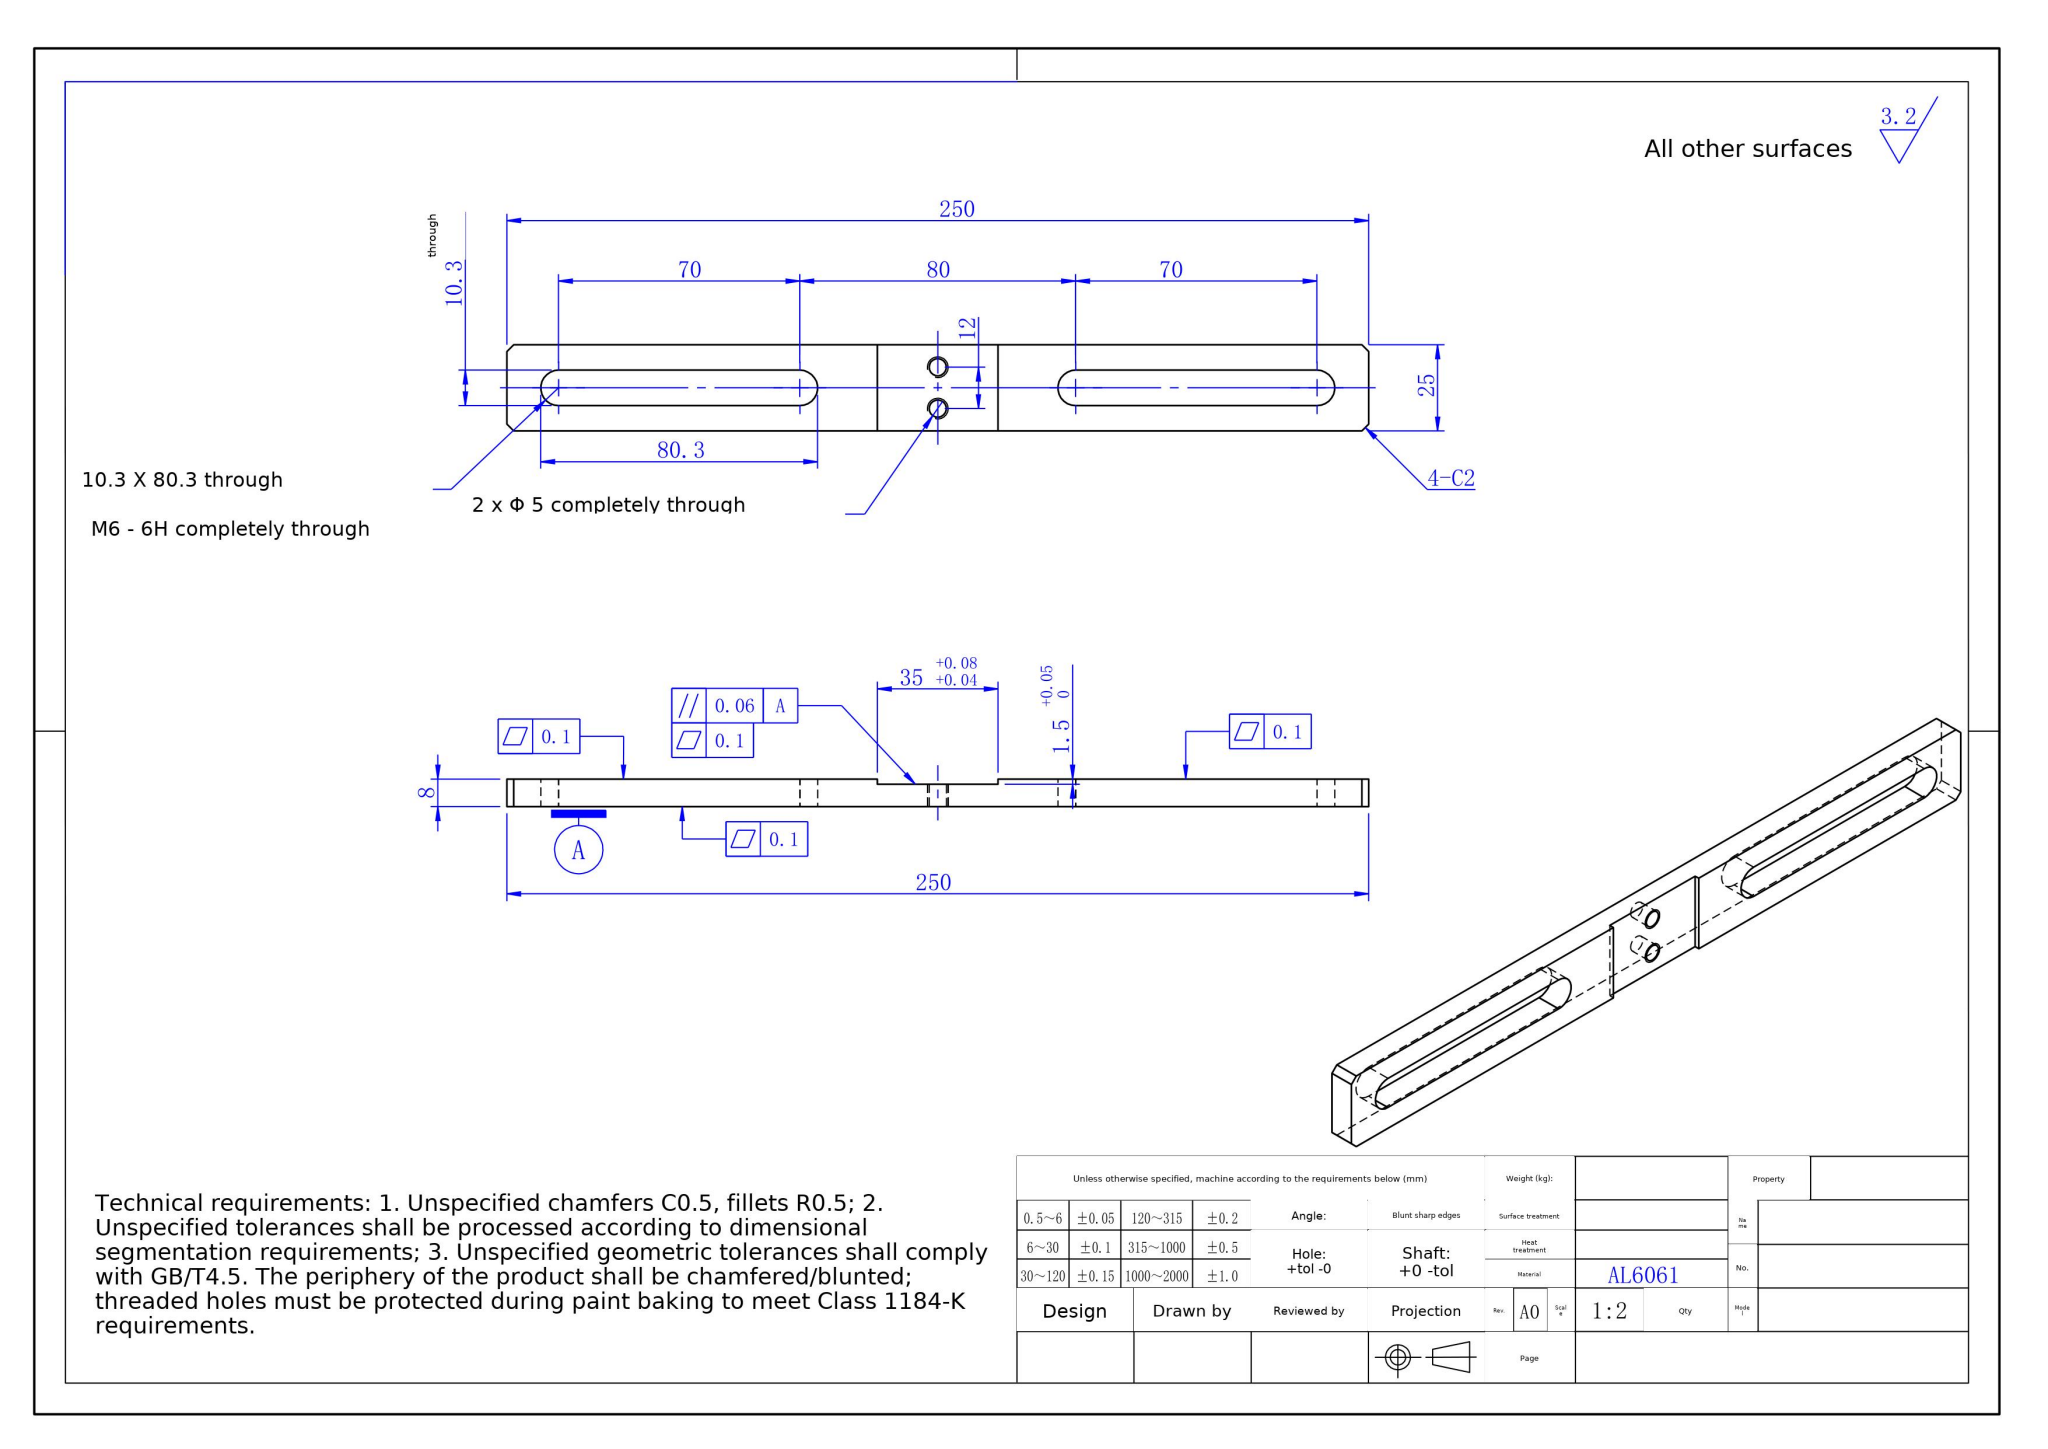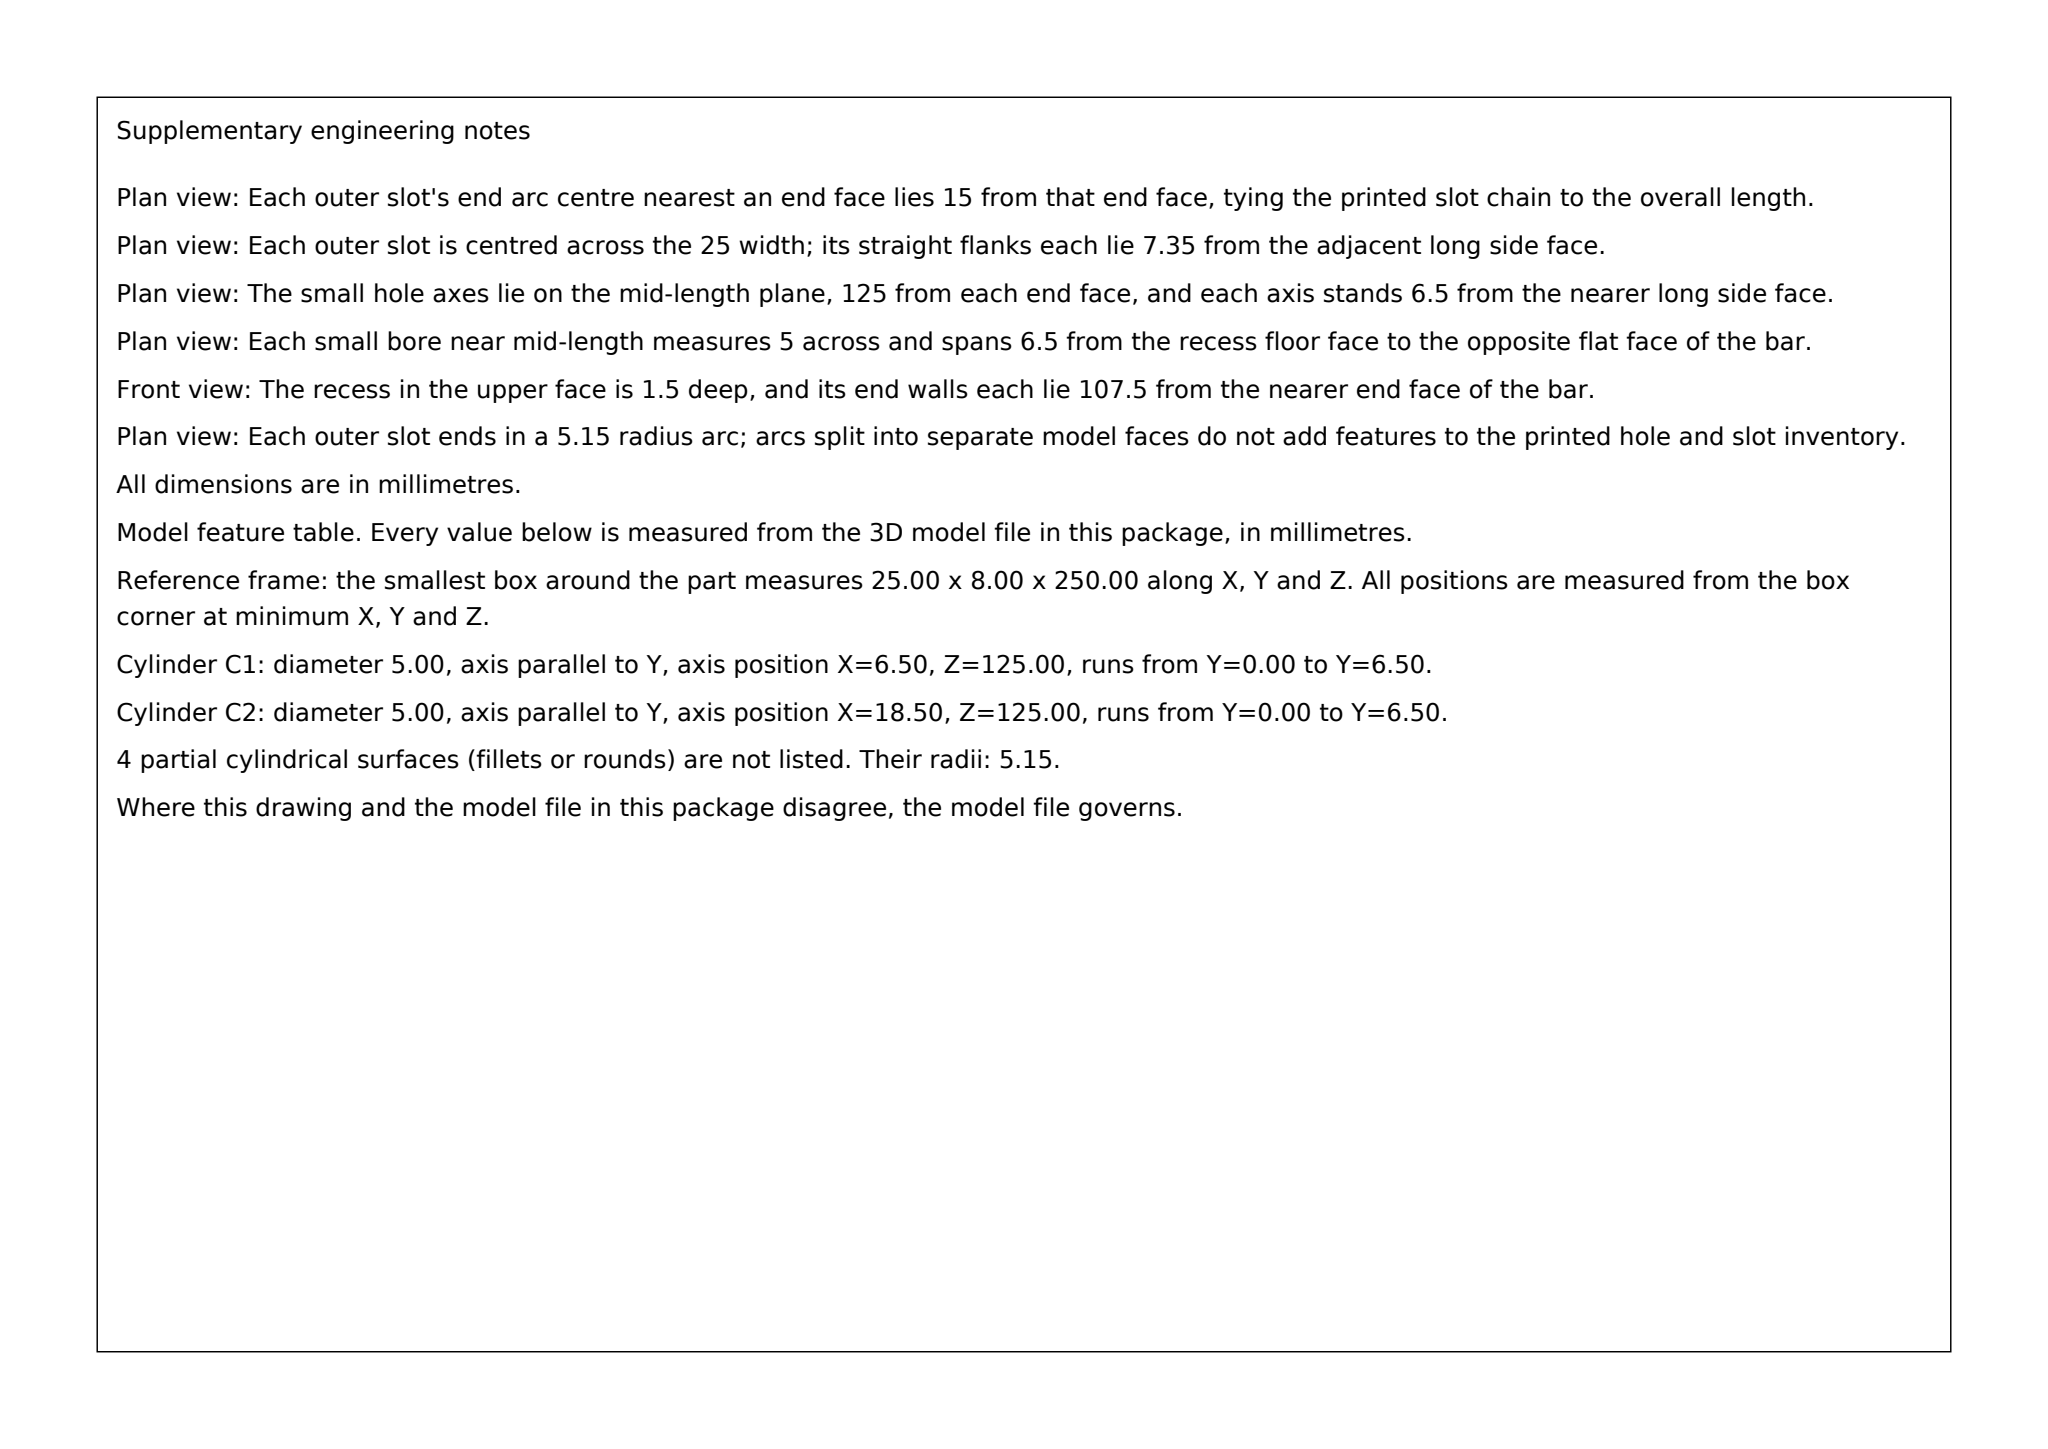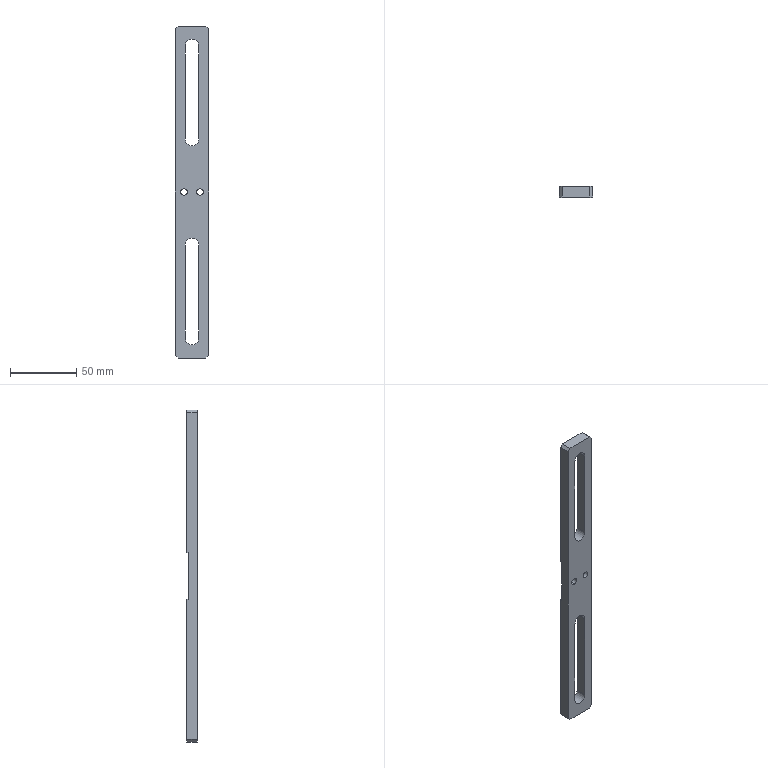Part | SolidWorks | mm | 1 solid | 28 faces | box 25 x 8 x 250 mm | volume 35499 mm3 | plane 18 | cylinder 10 | commonest cylinder face diameters 10.3 x6 5 x4
build123d program:
from build123d import *

# Parameters (mm, degrees)
SKETCH1_W           = 25
SKETCH1_H           = 250
BOSS_EXTRUDE1_DEPTH = 8
SKETCH2_W           = 25
SKETCH2_H           = 35
CUT_EXTRUDE1_DEPTH  = 1.5
M6_TAPPED_HOLE1_D   = 5
CUT_EXTRUDE2_DEPTH  = 10
CHAMFER1_SIZE       = 2


with BuildPart() as part:
    # Sketch1 → Boss-Extrude1 (new body)
    with BuildSketch(Plane(origin=(0, 0, 0), x_dir=(1, 0, 0), z_dir=(0, 1, 0))):
        Rectangle(SKETCH1_W, SKETCH1_H)
    extrude(amount=BOSS_EXTRUDE1_DEPTH)

    # Sketch2 → Cut-Extrude1 (cut)
    with BuildSketch(Plane(origin=(0, 8, 0), x_dir=(1, 0, 0), z_dir=(0, 1, 0))):
        Rectangle(SKETCH2_W, SKETCH2_H)
    extrude(amount=-CUT_EXTRUDE1_DEPTH, mode=Mode.SUBTRACT)

    # M6 Tapped Hole1 (through all)
    with Locations(Plane(origin=(0, 6.5, 0), x_dir=(1, 0, 0), z_dir=(0, 1, 0))):
        with Locations((-6, 0), (6, 0)):
            Hole(M6_TAPPED_HOLE1_D / 2)

    # Sketch5 → Cut-Extrude2 (cut)
    with BuildSketch(Plane(origin=(0, 8, 0), x_dir=(1, 0, 0), z_dir=(0, 1, 0))):
        with BuildLine():
            Line((5.15, -40), (5.15, -110))
            ThreePointArc((5.15, -110), (0, -115.15), (-5.15, -110))
            Line((-5.15, -110), (-5.15, -40))
            ThreePointArc((-5.15, -40), (0, -34.85), (5.15, -40))
        make_face()
        with BuildLine():
            Line((5.15, 40), (5.15, 110))
            ThreePointArc((5.15, 110), (0, 115.15), (-5.15, 110))
            Line((-5.15, 110), (-5.15, 40))
            ThreePointArc((-5.15, 40), (0, 34.85), (5.15, 40))
        make_face()
    extrude(amount=-CUT_EXTRUDE2_DEPTH, mode=Mode.SUBTRACT)

    # Chamfer1
    chamfer1_edges = [part.edges().sort_by_distance(p)[0] for p in [
        (12.5, 4, 125),
        (-12.5, 4, 125),
        (-12.5, 4, -125),
        (12.5, 4, -125),
    ]]
    chamfer(chamfer1_edges, length=CHAMFER1_SIZE)


solid = part.part
STEP:
#1=CARTESIAN_POINT('',(0.,0.,115.15));
#2=VERTEX_POINT('',#1);
#3=CARTESIAN_POINT('',(5.15,0.,110.));
#4=VERTEX_POINT('',#3);
#5=CARTESIAN_POINT('',(0.,0.,110.));
#6=DIRECTION('',(0.,1.,0.));
#7=DIRECTION('',(0.,0.,1.));
#8=AXIS2_PLACEMENT_3D('',#5,#6,#7);
#9=CIRCLE('',#8,5.15);
#10=EDGE_CURVE('',#2,#4,#9,.T.);
#11=ORIENTED_EDGE('',*,*,#10,.F.);
#12=CARTESIAN_POINT('',(0.,8.,115.15));
#13=VERTEX_POINT('',#12);
#14=CARTESIAN_POINT('',(0.,-2.,115.15));
#15=DIRECTION('',(0.,1.,0.));
#16=VECTOR('',#15,1000.);
#17=LINE('',#14,#16);
#18=EDGE_CURVE('',#2,#13,#17,.T.);
#19=ORIENTED_EDGE('',*,*,#18,.T.);
#20=CARTESIAN_POINT('',(5.15,8.,110.));
#21=VERTEX_POINT('',#20);
#22=CARTESIAN_POINT('',(0.,8.,110.));
#23=DIRECTION('',(0.,1.,0.));
#24=DIRECTION('',(0.,0.,1.));
#25=AXIS2_PLACEMENT_3D('',#22,#23,#24);
#26=CIRCLE('',#25,5.15);
#27=EDGE_CURVE('',#13,#21,#26,.T.);
#28=ORIENTED_EDGE('',*,*,#27,.T.);
#29=CARTESIAN_POINT('',(5.15,-2.,110.));
#30=DIRECTION('',(0.,1.,0.));
#31=VECTOR('',#30,1000.);
#32=LINE('',#29,#31);
#33=EDGE_CURVE('',#4,#21,#32,.T.);
#34=ORIENTED_EDGE('',*,*,#33,.F.);
#35=EDGE_LOOP('',(#11,#19,#28,#34));
#36=FACE_OUTER_BOUND('',#35,.T.);
#37=CARTESIAN_POINT('',(0.,-2.,110.));
#38=DIRECTION('',(0.,1.,0.));
#39=DIRECTION('',(0.,0.,1.));
#40=AXIS2_PLACEMENT_3D('',#37,#38,#39);
#41=CYLINDRICAL_SURFACE('',#40,5.15);
#42=ADVANCED_FACE('',(#36),#41,.F.);
#43=CARTESIAN_POINT('',(-0.,0.,-34.85));
#44=VERTEX_POINT('',#43);
#45=CARTESIAN_POINT('',(5.15,0.,-40.));
#46=VERTEX_POINT('',#45);
#47=CARTESIAN_POINT('',(-0.,0.,-40.));
#48=DIRECTION('',(0.,1.,0.));
#49=DIRECTION('',(0.,0.,1.));
#50=AXIS2_PLACEMENT_3D('',#47,#48,#49);
#51=CIRCLE('',#50,5.15);
#52=EDGE_CURVE('',#44,#46,#51,.T.);
#53=ORIENTED_EDGE('',*,*,#52,.F.);
#54=CARTESIAN_POINT('',(-0.,8.,-34.85));
#55=VERTEX_POINT('',#54);
#56=CARTESIAN_POINT('',(-0.,-2.,-34.85));
#57=DIRECTION('',(0.,1.,0.));
#58=VECTOR('',#57,1000.);
#59=LINE('',#56,#58);
#60=EDGE_CURVE('',#44,#55,#59,.T.);
#61=ORIENTED_EDGE('',*,*,#60,.T.);
#62=CARTESIAN_POINT('',(5.15,8.,-40.));
#63=VERTEX_POINT('',#62);
#64=CARTESIAN_POINT('',(-0.,8.,-40.));
#65=DIRECTION('',(0.,1.,0.));
#66=DIRECTION('',(0.,0.,-1.));
#67=AXIS2_PLACEMENT_3D('',#64,#65,#66);
#68=CIRCLE('',#67,5.15);
#69=EDGE_CURVE('',#55,#63,#68,.T.);
#70=ORIENTED_EDGE('',*,*,#69,.T.);
#71=CARTESIAN_POINT('',(5.15,-2.,-40.));
#72=DIRECTION('',(0.,1.,0.));
#73=VECTOR('',#72,1000.);
#74=LINE('',#71,#73);
#75=EDGE_CURVE('',#46,#63,#74,.T.);
#76=ORIENTED_EDGE('',*,*,#75,.F.);
#77=EDGE_LOOP('',(#53,#61,#70,#76));
#78=FACE_OUTER_BOUND('',#77,.T.);
#79=CARTESIAN_POINT('',(-0.,-2.,-40.));
#80=DIRECTION('',(0.,1.,0.));
#81=DIRECTION('',(0.,0.,1.));
#82=AXIS2_PLACEMENT_3D('',#79,#80,#81);
#83=CYLINDRICAL_SURFACE('',#82,5.15);
#84=ADVANCED_FACE('',(#78),#83,.F.);
#85=CARTESIAN_POINT('',(-6.,0.,-2.5));
#86=VERTEX_POINT('',#85);
#87=CARTESIAN_POINT('',(-6.,0.,2.5));
#88=VERTEX_POINT('',#87);
#89=CARTESIAN_POINT('',(-6.,0.,0.));
#90=DIRECTION('',(0.,1.,0.));
#91=DIRECTION('',(0.,0.,1.));
#92=AXIS2_PLACEMENT_3D('',#89,#90,#91);
#93=CIRCLE('',#92,2.5);
#94=EDGE_CURVE('',#86,#88,#93,.T.);
#95=ORIENTED_EDGE('',*,*,#94,.F.);
#96=CARTESIAN_POINT('',(-6.,6.5,-2.5));
#97=VERTEX_POINT('',#96);
#98=CARTESIAN_POINT('',(-6.,6.5,-2.5));
#99=DIRECTION('',(0.,1.,0.));
#100=VECTOR('',#99,1000.);
#101=LINE('',#98,#100);
#102=EDGE_CURVE('',#86,#97,#101,.T.);
#103=ORIENTED_EDGE('',*,*,#102,.T.);
#104=CARTESIAN_POINT('',(-6.,6.5,2.5));
#105=VERTEX_POINT('',#104);
#106=CARTESIAN_POINT('',(-6.,6.5,0.));
#107=DIRECTION('',(0.,1.,0.));
#108=DIRECTION('',(0.,0.,1.));
#109=AXIS2_PLACEMENT_3D('',#106,#107,#108);
#110=CIRCLE('',#109,2.5);
#111=EDGE_CURVE('',#97,#105,#110,.T.);
#112=ORIENTED_EDGE('',*,*,#111,.T.);
#113=CARTESIAN_POINT('',(-6.,6.5,2.5));
#114=DIRECTION('',(0.,1.,0.));
#115=VECTOR('',#114,1000.);
#116=LINE('',#113,#115);
#117=EDGE_CURVE('',#88,#105,#116,.T.);
#118=ORIENTED_EDGE('',*,*,#117,.F.);
#119=EDGE_LOOP('',(#95,#103,#112,#118));
#120=FACE_OUTER_BOUND('',#119,.T.);
#121=CARTESIAN_POINT('',(-6.,6.5,0.));
#122=DIRECTION('',(0.,1.,0.));
#123=DIRECTION('',(0.,0.,1.));
#124=AXIS2_PLACEMENT_3D('',#121,#122,#123);
#125=CYLINDRICAL_SURFACE('',#124,2.5);
#126=ADVANCED_FACE('',(#120),#125,.F.);
#127=CARTESIAN_POINT('',(6.,0.,-2.5));
#128=VERTEX_POINT('',#127);
#129=CARTESIAN_POINT('',(6.,0.,2.5));
#130=VERTEX_POINT('',#129);
#131=CARTESIAN_POINT('',(6.,0.,0.));
#132=DIRECTION('',(0.,1.,0.));
#133=DIRECTION('',(0.,0.,1.));
#134=AXIS2_PLACEMENT_3D('',#131,#132,#133);
#135=CIRCLE('',#134,2.5);
#136=EDGE_CURVE('',#128,#130,#135,.T.);
#137=ORIENTED_EDGE('',*,*,#136,.F.);
#138=CARTESIAN_POINT('',(6.,6.5,-2.5));
#139=VERTEX_POINT('',#138);
#140=CARTESIAN_POINT('',(6.,6.5,-2.5));
#141=DIRECTION('',(0.,1.,0.));
#142=VECTOR('',#141,1000.);
#143=LINE('',#140,#142);
#144=EDGE_CURVE('',#128,#139,#143,.T.);
#145=ORIENTED_EDGE('',*,*,#144,.T.);
#146=CARTESIAN_POINT('',(6.,6.5,2.5));
#147=VERTEX_POINT('',#146);
#148=CARTESIAN_POINT('',(6.,6.5,0.));
#149=DIRECTION('',(0.,1.,0.));
#150=DIRECTION('',(0.,0.,1.));
#151=AXIS2_PLACEMENT_3D('',#148,#149,#150);
#152=CIRCLE('',#151,2.5);
#153=EDGE_CURVE('',#139,#147,#152,.T.);
#154=ORIENTED_EDGE('',*,*,#153,.T.);
#155=CARTESIAN_POINT('',(6.,6.5,2.5));
#156=DIRECTION('',(0.,1.,0.));
#157=VECTOR('',#156,1000.);
#158=LINE('',#155,#157);
#159=EDGE_CURVE('',#130,#147,#158,.T.);
#160=ORIENTED_EDGE('',*,*,#159,.F.);
#161=EDGE_LOOP('',(#137,#145,#154,#160));
#162=FACE_OUTER_BOUND('',#161,.T.);
#163=CARTESIAN_POINT('',(6.,6.5,0.));
#164=DIRECTION('',(0.,1.,0.));
#165=DIRECTION('',(0.,0.,1.));
#166=AXIS2_PLACEMENT_3D('',#163,#164,#165);
#167=CYLINDRICAL_SURFACE('',#166,2.5);
#168=ADVANCED_FACE('',(#162),#167,.F.);
#169=CARTESIAN_POINT('',(5.15,8.,40.));
#170=VERTEX_POINT('',#169);
#171=CARTESIAN_POINT('',(-5.15,8.,40.));
#172=VERTEX_POINT('',#171);
#173=CARTESIAN_POINT('',(0.,8.,40.));
#174=DIRECTION('',(0.,1.,0.));
#175=DIRECTION('',(0.,0.,1.));
#176=AXIS2_PLACEMENT_3D('',#173,#174,#175);
#177=CIRCLE('',#176,5.15);
#178=EDGE_CURVE('',#170,#172,#177,.T.);
#179=ORIENTED_EDGE('',*,*,#178,.F.);
#180=CARTESIAN_POINT('',(5.15,8.,40.));
#181=DIRECTION('',(-0.,0.,-1.));
#182=VECTOR('',#181,1000.);
#183=LINE('',#180,#182);
#184=EDGE_CURVE('',#21,#170,#183,.T.);
#185=ORIENTED_EDGE('',*,*,#184,.F.);
#186=ORIENTED_EDGE('',*,*,#27,.F.);
#187=CARTESIAN_POINT('',(-5.15,8.,110.));
#188=VERTEX_POINT('',#187);
#189=CARTESIAN_POINT('',(0.,8.,110.));
#190=DIRECTION('',(0.,1.,0.));
#191=DIRECTION('',(0.,0.,1.));
#192=AXIS2_PLACEMENT_3D('',#189,#190,#191);
#193=CIRCLE('',#192,5.15);
#194=EDGE_CURVE('',#188,#13,#193,.T.);
#195=ORIENTED_EDGE('',*,*,#194,.F.);
#196=CARTESIAN_POINT('',(-5.15,8.,40.));
#197=DIRECTION('',(-0.,0.,1.));
#198=VECTOR('',#197,1000.);
#199=LINE('',#196,#198);
#200=EDGE_CURVE('',#172,#188,#199,.T.);
#201=ORIENTED_EDGE('',*,*,#200,.F.);
#202=EDGE_LOOP('',(#179,#185,#186,#195,#201));
#203=FACE_BOUND('',#202,.T.);
#204=CARTESIAN_POINT('',(-12.5,8.,17.5));
#205=VERTEX_POINT('',#204);
#206=CARTESIAN_POINT('',(-12.5,8.,123.));
#207=VERTEX_POINT('',#206);
#208=CARTESIAN_POINT('',(-12.5,8.,-125.));
#209=DIRECTION('',(0.,0.,1.));
#210=VECTOR('',#209,1000.);
#211=LINE('',#208,#210);
#212=EDGE_CURVE('',#205,#207,#211,.T.);
#213=ORIENTED_EDGE('',*,*,#212,.T.);
#214=CARTESIAN_POINT('',(-10.5,8.,125.));
#215=VERTEX_POINT('',#214);
#216=CARTESIAN_POINT('',(-67.75,8.,67.75));
#217=DIRECTION('',(0.7071,0.,0.7071));
#218=VECTOR('',#217,1000.);
#219=LINE('',#216,#218);
#220=EDGE_CURVE('',#207,#215,#219,.T.);
#221=ORIENTED_EDGE('',*,*,#220,.T.);
#222=CARTESIAN_POINT('',(10.5,8.,125.));
#223=VERTEX_POINT('',#222);
#224=CARTESIAN_POINT('',(-12.5,8.,125.));
#225=DIRECTION('',(1.,0.,0.));
#226=VECTOR('',#225,1000.);
#227=LINE('',#224,#226);
#228=EDGE_CURVE('',#215,#223,#227,.T.);
#229=ORIENTED_EDGE('',*,*,#228,.T.);
#230=CARTESIAN_POINT('',(12.5,8.,123.));
#231=VERTEX_POINT('',#230);
#232=CARTESIAN_POINT('',(67.75,8.,67.75));
#233=DIRECTION('',(0.7071,0.,-0.7071));
#234=VECTOR('',#233,1000.);
#235=LINE('',#232,#234);
#236=EDGE_CURVE('',#223,#231,#235,.T.);
#237=ORIENTED_EDGE('',*,*,#236,.T.);
#238=CARTESIAN_POINT('',(12.5,8.,17.5));
#239=VERTEX_POINT('',#238);
#240=CARTESIAN_POINT('',(12.5,8.,-125.));
#241=DIRECTION('',(-0.,0.,-1.));
#242=VECTOR('',#241,1000.);
#243=LINE('',#240,#242);
#244=EDGE_CURVE('',#231,#239,#243,.T.);
#245=ORIENTED_EDGE('',*,*,#244,.T.);
#246=CARTESIAN_POINT('',(-12.5,8.,17.5));
#247=DIRECTION('',(1.,0.,0.));
#248=VECTOR('',#247,1000.);
#249=LINE('',#246,#248);
#250=EDGE_CURVE('',#205,#239,#249,.T.);
#251=ORIENTED_EDGE('',*,*,#250,.F.);
#252=EDGE_LOOP('',(#213,#221,#229,#237,#245,#251));
#253=FACE_OUTER_BOUND('',#252,.T.);
#254=CARTESIAN_POINT('',(0.,8.,0.));
#255=DIRECTION('',(0.,1.,0.));
#256=DIRECTION('',(0.,0.,1.));
#257=AXIS2_PLACEMENT_3D('',#254,#255,#256);
#258=PLANE('',#257);
#259=ADVANCED_FACE('',(#203,#253),#258,.T.);
#260=CARTESIAN_POINT('',(12.5,0.,123.));
#261=VERTEX_POINT('',#260);
#262=CARTESIAN_POINT('',(12.5,0.,-123.));
#263=VERTEX_POINT('',#262);
#264=CARTESIAN_POINT('',(12.5,0.,-125.));
#265=DIRECTION('',(-0.,0.,-1.));
#266=VECTOR('',#265,1000.);
#267=LINE('',#264,#266);
#268=EDGE_CURVE('',#261,#263,#267,.T.);
#269=ORIENTED_EDGE('',*,*,#268,.T.);
#270=CARTESIAN_POINT('',(12.5,8.,-123.));
#271=VERTEX_POINT('',#270);
#272=CARTESIAN_POINT('',(12.5,8.,-123.));
#273=DIRECTION('',(0.,1.,0.));
#274=VECTOR('',#273,1000.);
#275=LINE('',#272,#274);
#276=EDGE_CURVE('',#263,#271,#275,.T.);
#277=ORIENTED_EDGE('',*,*,#276,.T.);
#278=CARTESIAN_POINT('',(12.5,8.,-17.5));
#279=VERTEX_POINT('',#278);
#280=CARTESIAN_POINT('',(12.5,8.,-125.));
#281=DIRECTION('',(-0.,0.,-1.));
#282=VECTOR('',#281,1000.);
#283=LINE('',#280,#282);
#284=EDGE_CURVE('',#279,#271,#283,.T.);
#285=ORIENTED_EDGE('',*,*,#284,.F.);
#286=CARTESIAN_POINT('',(12.5,6.5,-17.5));
#287=VERTEX_POINT('',#286);
#288=CARTESIAN_POINT('',(12.5,6.5,-17.5));
#289=DIRECTION('',(0.,1.,0.));
#290=VECTOR('',#289,1000.);
#291=LINE('',#288,#290);
#292=EDGE_CURVE('',#287,#279,#291,.T.);
#293=ORIENTED_EDGE('',*,*,#292,.F.);
#294=CARTESIAN_POINT('',(12.5,6.5,17.5));
#295=VERTEX_POINT('',#294);
#296=CARTESIAN_POINT('',(12.5,6.5,-17.5));
#297=DIRECTION('',(0.,0.,-1.));
#298=VECTOR('',#297,1000.);
#299=LINE('',#296,#298);
#300=EDGE_CURVE('',#295,#287,#299,.T.);
#301=ORIENTED_EDGE('',*,*,#300,.F.);
#302=CARTESIAN_POINT('',(12.5,6.5,17.5));
#303=DIRECTION('',(0.,1.,0.));
#304=VECTOR('',#303,1000.);
#305=LINE('',#302,#304);
#306=EDGE_CURVE('',#295,#239,#305,.T.);
#307=ORIENTED_EDGE('',*,*,#306,.T.);
#308=ORIENTED_EDGE('',*,*,#244,.F.);
#309=CARTESIAN_POINT('',(12.5,8.,123.));
#310=DIRECTION('',(0.,-1.,0.));
#311=VECTOR('',#310,1000.);
#312=LINE('',#309,#311);
#313=EDGE_CURVE('',#231,#261,#312,.T.);
#314=ORIENTED_EDGE('',*,*,#313,.T.);
#315=EDGE_LOOP('',(#269,#277,#285,#293,#301,#307,#308,#314));
#316=FACE_OUTER_BOUND('',#315,.T.);
#317=CARTESIAN_POINT('',(12.5,8.,-125.));
#318=DIRECTION('',(-1.,0.,0.));
#319=DIRECTION('',(0.,0.,1.));
#320=AXIS2_PLACEMENT_3D('',#317,#318,#319);
#321=PLANE('',#320);
#322=ADVANCED_FACE('',(#316),#321,.F.);
#323=CARTESIAN_POINT('',(10.5,0.,-125.));
#324=VERTEX_POINT('',#323);
#325=CARTESIAN_POINT('',(-10.5,0.,-125.));
#326=VERTEX_POINT('',#325);
#327=CARTESIAN_POINT('',(-12.5,0.,-125.));
#328=DIRECTION('',(-1.,0.,0.));
#329=VECTOR('',#328,1000.);
#330=LINE('',#327,#329);
#331=EDGE_CURVE('',#324,#326,#330,.T.);
#332=ORIENTED_EDGE('',*,*,#331,.T.);
#333=CARTESIAN_POINT('',(-10.5,8.,-125.));
#334=VERTEX_POINT('',#333);
#335=CARTESIAN_POINT('',(-10.5,8.,-125.));
#336=DIRECTION('',(0.,1.,0.));
#337=VECTOR('',#336,1000.);
#338=LINE('',#335,#337);
#339=EDGE_CURVE('',#326,#334,#338,.T.);
#340=ORIENTED_EDGE('',*,*,#339,.T.);
#341=CARTESIAN_POINT('',(10.5,8.,-125.));
#342=VERTEX_POINT('',#341);
#343=CARTESIAN_POINT('',(-12.5,8.,-125.));
#344=DIRECTION('',(-1.,0.,0.));
#345=VECTOR('',#344,1000.);
#346=LINE('',#343,#345);
#347=EDGE_CURVE('',#342,#334,#346,.T.);
#348=ORIENTED_EDGE('',*,*,#347,.F.);
#349=CARTESIAN_POINT('',(10.5,8.,-125.));
#350=DIRECTION('',(0.,-1.,0.));
#351=VECTOR('',#350,1000.);
#352=LINE('',#349,#351);
#353=EDGE_CURVE('',#342,#324,#352,.T.);
#354=ORIENTED_EDGE('',*,*,#353,.T.);
#355=EDGE_LOOP('',(#332,#340,#348,#354));
#356=FACE_OUTER_BOUND('',#355,.T.);
#357=CARTESIAN_POINT('',(-12.5,8.,-125.));
#358=DIRECTION('',(0.,0.,1.));
#359=DIRECTION('',(1.,0.,0.));
#360=AXIS2_PLACEMENT_3D('',#357,#358,#359);
#361=PLANE('',#360);
#362=ADVANCED_FACE('',(#356),#361,.F.);
#363=CARTESIAN_POINT('',(-12.5,8.,-123.));
#364=VERTEX_POINT('',#363);
#365=CARTESIAN_POINT('',(-12.5,8.,-17.5));
#366=VERTEX_POINT('',#365);
#367=CARTESIAN_POINT('',(-12.5,8.,-125.));
#368=DIRECTION('',(0.,0.,1.));
#369=VECTOR('',#368,1000.);
#370=LINE('',#367,#369);
#371=EDGE_CURVE('',#364,#366,#370,.T.);
#372=ORIENTED_EDGE('',*,*,#371,.F.);
#373=CARTESIAN_POINT('',(-12.5,0.,-123.));
#374=VERTEX_POINT('',#373);
#375=CARTESIAN_POINT('',(-12.5,8.,-123.));
#376=DIRECTION('',(0.,-1.,0.));
#377=VECTOR('',#376,1000.);
#378=LINE('',#375,#377);
#379=EDGE_CURVE('',#364,#374,#378,.T.);
#380=ORIENTED_EDGE('',*,*,#379,.T.);
#381=CARTESIAN_POINT('',(-12.5,0.,123.));
#382=VERTEX_POINT('',#381);
#383=CARTESIAN_POINT('',(-12.5,0.,-125.));
#384=DIRECTION('',(0.,0.,1.));
#385=VECTOR('',#384,1000.);
#386=LINE('',#383,#385);
#387=EDGE_CURVE('',#374,#382,#386,.T.);
#388=ORIENTED_EDGE('',*,*,#387,.T.);
#389=CARTESIAN_POINT('',(-12.5,8.,123.));
#390=DIRECTION('',(0.,1.,0.));
#391=VECTOR('',#390,1000.);
#392=LINE('',#389,#391);
#393=EDGE_CURVE('',#382,#207,#392,.T.);
#394=ORIENTED_EDGE('',*,*,#393,.T.);
#395=ORIENTED_EDGE('',*,*,#212,.F.);
#396=CARTESIAN_POINT('',(-12.5,6.5,17.5));
#397=VERTEX_POINT('',#396);
#398=CARTESIAN_POINT('',(-12.5,6.5,17.5));
#399=DIRECTION('',(0.,1.,0.));
#400=VECTOR('',#399,1000.);
#401=LINE('',#398,#400);
#402=EDGE_CURVE('',#397,#205,#401,.T.);
#403=ORIENTED_EDGE('',*,*,#402,.F.);
#404=CARTESIAN_POINT('',(-12.5,6.5,-17.5));
#405=VERTEX_POINT('',#404);
#406=CARTESIAN_POINT('',(-12.5,6.5,-17.5));
#407=DIRECTION('',(0.,0.,1.));
#408=VECTOR('',#407,1000.);
#409=LINE('',#406,#408);
#410=EDGE_CURVE('',#405,#397,#409,.T.);
#411=ORIENTED_EDGE('',*,*,#410,.F.);
#412=CARTESIAN_POINT('',(-12.5,6.5,-17.5));
#413=DIRECTION('',(0.,1.,0.));
#414=VECTOR('',#413,1000.);
#415=LINE('',#412,#414);
#416=EDGE_CURVE('',#405,#366,#415,.T.);
#417=ORIENTED_EDGE('',*,*,#416,.T.);
#418=EDGE_LOOP('',(#372,#380,#388,#394,#395,#403,#411,#417));
#419=FACE_OUTER_BOUND('',#418,.T.);
#420=CARTESIAN_POINT('',(-12.5,8.,-125.));
#421=DIRECTION('',(1.,0.,-0.));
#422=DIRECTION('',(-0.,0.,-1.));
#423=AXIS2_PLACEMENT_3D('',#420,#421,#422);
#424=PLANE('',#423);
#425=ADVANCED_FACE('',(#419),#424,.F.);
#426=ORIENTED_EDGE('',*,*,#228,.F.);
#427=CARTESIAN_POINT('',(-10.5,0.,125.));
#428=VERTEX_POINT('',#427);
#429=CARTESIAN_POINT('',(-10.5,8.,125.));
#430=DIRECTION('',(0.,-1.,0.));
#431=VECTOR('',#430,1000.);
#432=LINE('',#429,#431);
#433=EDGE_CURVE('',#215,#428,#432,.T.);
#434=ORIENTED_EDGE('',*,*,#433,.T.);
#435=CARTESIAN_POINT('',(10.5,0.,125.));
#436=VERTEX_POINT('',#435);
#437=CARTESIAN_POINT('',(-12.5,0.,125.));
#438=DIRECTION('',(1.,0.,0.));
#439=VECTOR('',#438,1000.);
#440=LINE('',#437,#439);
#441=EDGE_CURVE('',#428,#436,#440,.T.);
#442=ORIENTED_EDGE('',*,*,#441,.T.);
#443=CARTESIAN_POINT('',(10.5,8.,125.));
#444=DIRECTION('',(0.,1.,0.));
#445=VECTOR('',#444,1000.);
#446=LINE('',#443,#445);
#447=EDGE_CURVE('',#436,#223,#446,.T.);
#448=ORIENTED_EDGE('',*,*,#447,.T.);
#449=EDGE_LOOP('',(#426,#434,#442,#448));
#450=FACE_OUTER_BOUND('',#449,.T.);
#451=CARTESIAN_POINT('',(-12.5,8.,125.));
#452=DIRECTION('',(0.,0.,-1.));
#453=DIRECTION('',(-1.,0.,0.));
#454=AXIS2_PLACEMENT_3D('',#451,#452,#453);
#455=PLANE('',#454);
#456=ADVANCED_FACE('',(#450),#455,.F.);
#457=CARTESIAN_POINT('',(-5.15,8.,-40.));
#458=VERTEX_POINT('',#457);
#459=CARTESIAN_POINT('',(-0.,8.,-40.));
#460=DIRECTION('',(0.,1.,0.));
#461=DIRECTION('',(0.,0.,-1.));
#462=AXIS2_PLACEMENT_3D('',#459,#460,#461);
#463=CIRCLE('',#462,5.15);
#464=EDGE_CURVE('',#458,#55,#463,.T.);
#465=ORIENTED_EDGE('',*,*,#464,.F.);
#466=CARTESIAN_POINT('',(-5.15,8.,-110.));
#467=VERTEX_POINT('',#466);
#468=CARTESIAN_POINT('',(-5.15,8.,-40.));
#469=DIRECTION('',(0.,0.,1.));
#470=VECTOR('',#469,1000.);
#471=LINE('',#468,#470);
#472=EDGE_CURVE('',#467,#458,#471,.T.);
#473=ORIENTED_EDGE('',*,*,#472,.F.);
#474=CARTESIAN_POINT('',(5.15,8.,-110.));
#475=VERTEX_POINT('',#474);
#476=CARTESIAN_POINT('',(-0.,8.,-110.));
#477=DIRECTION('',(0.,1.,0.));
#478=DIRECTION('',(0.,0.,-1.));
#479=AXIS2_PLACEMENT_3D('',#476,#477,#478);
#480=CIRCLE('',#479,5.15);
#481=EDGE_CURVE('',#475,#467,#480,.T.);
#482=ORIENTED_EDGE('',*,*,#481,.F.);
#483=CARTESIAN_POINT('',(5.15,8.,-40.));
#484=DIRECTION('',(-0.,0.,-1.));
#485=VECTOR('',#484,1000.);
#486=LINE('',#483,#485);
#487=EDGE_CURVE('',#63,#475,#486,.T.);
#488=ORIENTED_EDGE('',*,*,#487,.F.);
#489=ORIENTED_EDGE('',*,*,#69,.F.);
#490=EDGE_LOOP('',(#465,#473,#482,#488,#489));
#491=FACE_BOUND('',#490,.T.);
#492=ORIENTED_EDGE('',*,*,#347,.T.);
#493=CARTESIAN_POINT('',(-67.75,8.,-67.75));
#494=DIRECTION('',(-0.7071,0.,0.7071));
#495=VECTOR('',#494,1000.);
#496=LINE('',#493,#495);
#497=EDGE_CURVE('',#334,#364,#496,.T.);
#498=ORIENTED_EDGE('',*,*,#497,.T.);
#499=ORIENTED_EDGE('',*,*,#371,.T.);
#500=CARTESIAN_POINT('',(-12.5,8.,-17.5));
#501=DIRECTION('',(-1.,0.,0.));
#502=VECTOR('',#501,1000.);
#503=LINE('',#500,#502);
#504=EDGE_CURVE('',#279,#366,#503,.T.);
#505=ORIENTED_EDGE('',*,*,#504,.F.);
#506=ORIENTED_EDGE('',*,*,#284,.T.);
#507=CARTESIAN_POINT('',(67.75,8.,-67.75));
#508=DIRECTION('',(-0.7071,0.,-0.7071));
#509=VECTOR('',#508,1000.);
#510=LINE('',#507,#509);
#511=EDGE_CURVE('',#271,#342,#510,.T.);
#512=ORIENTED_EDGE('',*,*,#511,.T.);
#513=EDGE_LOOP('',(#492,#498,#499,#505,#506,#512));
#514=FACE_OUTER_BOUND('',#513,.T.);
#515=CARTESIAN_POINT('',(0.,8.,0.));
#516=DIRECTION('',(0.,1.,0.));
#517=DIRECTION('',(0.,0.,1.));
#518=AXIS2_PLACEMENT_3D('',#515,#516,#517);
#519=PLANE('',#518);
#520=ADVANCED_FACE('',(#491,#514),#519,.T.);
#521=CARTESIAN_POINT('',(5.15,0.,40.));
#522=VERTEX_POINT('',#521);
#523=CARTESIAN_POINT('',(5.15,0.,-0.));
#524=DIRECTION('',(-0.,0.,-1.));
#525=VECTOR('',#524,1000.);
#526=LINE('',#523,#525);
#527=EDGE_CURVE('',#4,#522,#526,.T.);
#528=ORIENTED_EDGE('',*,*,#527,.T.);
#529=CARTESIAN_POINT('',(-5.15,0.,40.));
#530=VERTEX_POINT('',#529);
#531=CARTESIAN_POINT('',(0.,0.,40.));
#532=DIRECTION('',(0.,1.,0.));
#533=DIRECTION('',(0.,0.,1.));
#534=AXIS2_PLACEMENT_3D('',#531,#532,#533);
#535=CIRCLE('',#534,5.15);
#536=EDGE_CURVE('',#522,#530,#535,.T.);
#537=ORIENTED_EDGE('',*,*,#536,.T.);
#538=CARTESIAN_POINT('',(-5.15,0.,110.));
#539=VERTEX_POINT('',#538);
#540=CARTESIAN_POINT('',(-5.15,0.,-0.));
#541=DIRECTION('',(-0.,0.,1.));
#542=VECTOR('',#541,1000.);
#543=LINE('',#540,#542);
#544=EDGE_CURVE('',#530,#539,#543,.T.);
#545=ORIENTED_EDGE('',*,*,#544,.T.);
#546=CARTESIAN_POINT('',(0.,0.,110.));
#547=DIRECTION('',(0.,1.,0.));
#548=DIRECTION('',(0.,0.,1.));
#549=AXIS2_PLACEMENT_3D('',#546,#547,#548);
#550=CIRCLE('',#549,5.15);
#551=EDGE_CURVE('',#539,#2,#550,.T.);
#552=ORIENTED_EDGE('',*,*,#551,.T.);
#553=ORIENTED_EDGE('',*,*,#10,.T.);
#554=EDGE_LOOP('',(#528,#537,#545,#552,#553));
#555=FACE_BOUND('',#554,.T.);
#556=CARTESIAN_POINT('',(-5.15,0.,-110.));
#557=VERTEX_POINT('',#556);
#558=CARTESIAN_POINT('',(-5.15,0.,-40.));
#559=VERTEX_POINT('',#558);
#560=CARTESIAN_POINT('',(-5.15,0.,0.));
#561=DIRECTION('',(0.,0.,1.));
#562=VECTOR('',#561,1000.);
#563=LINE('',#560,#562);
#564=EDGE_CURVE('',#557,#559,#563,.T.);
#565=ORIENTED_EDGE('',*,*,#564,.T.);
#566=CARTESIAN_POINT('',(-0.,0.,-40.));
#567=DIRECTION('',(0.,1.,0.));
#568=DIRECTION('',(0.,0.,1.));
#569=AXIS2_PLACEMENT_3D('',#566,#567,#568);
#570=CIRCLE('',#569,5.15);
#571=EDGE_CURVE('',#559,#44,#570,.T.);
#572=ORIENTED_EDGE('',*,*,#571,.T.);
#573=ORIENTED_EDGE('',*,*,#52,.T.);
#574=CARTESIAN_POINT('',(5.15,0.,-110.));
#575=VERTEX_POINT('',#574);
#576=CARTESIAN_POINT('',(5.15,0.,-0.));
#577=DIRECTION('',(-0.,0.,-1.));
#578=VECTOR('',#577,1000.);
#579=LINE('',#576,#578);
#580=EDGE_CURVE('',#46,#575,#579,.T.);
#581=ORIENTED_EDGE('',*,*,#580,.T.);
#582=CARTESIAN_POINT('',(-0.,0.,-110.));
#583=DIRECTION('',(0.,1.,0.));
#584=DIRECTION('',(0.,0.,1.));
#585=AXIS2_PLACEMENT_3D('',#582,#583,#584);
#586=CIRCLE('',#585,5.15);
#587=EDGE_CURVE('',#575,#557,#586,.T.);
#588=ORIENTED_EDGE('',*,*,#587,.T.);
#589=EDGE_LOOP('',(#565,#572,#573,#581,#588));
#590=FACE_BOUND('',#589,.T.);
#591=CARTESIAN_POINT('',(-6.,0.,0.));
#592=DIRECTION('',(0.,1.,0.));
#593=DIRECTION('',(0.,0.,1.));
#594=AXIS2_PLACEMENT_3D('',#591,#592,#593);
#595=CIRCLE('',#594,2.5);
#596=EDGE_CURVE('',#88,#86,#595,.T.);
#597=ORIENTED_EDGE('',*,*,#596,.T.);
#598=ORIENTED_EDGE('',*,*,#94,.T.);
#599=EDGE_LOOP('',(#597,#598));
#600=FACE_BOUND('',#599,.T.);
#601=CARTESIAN_POINT('',(6.,0.,0.));
#602=DIRECTION('',(0.,1.,0.));
#603=DIRECTION('',(0.,0.,1.));
#604=AXIS2_PLACEMENT_3D('',#601,#602,#603);
#605=CIRCLE('',#604,2.5);
#606=EDGE_CURVE('',#130,#128,#605,.T.);
#607=ORIENTED_EDGE('',*,*,#606,.T.);
#608=ORIENTED_EDGE('',*,*,#136,.T.);
#609=EDGE_LOOP('',(#607,#608));
#610=FACE_BOUND('',#609,.T.);
#611=ORIENTED_EDGE('',*,*,#387,.F.);
#612=CARTESIAN_POINT('',(-12.5,0.,-123.));
#613=DIRECTION('',(0.7071,0.,-0.7071));
#614=VECTOR('',#613,1000.);
#615=LINE('',#612,#614);
#616=EDGE_CURVE('',#374,#326,#615,.T.);
#617=ORIENTED_EDGE('',*,*,#616,.T.);
#618=ORIENTED_EDGE('',*,*,#331,.F.);
#619=CARTESIAN_POINT('',(10.5,0.,-125.));
#620=DIRECTION('',(0.7071,0.,0.7071));
#621=VECTOR('',#620,1000.);
#622=LINE('',#619,#621);
#623=EDGE_CURVE('',#324,#263,#622,.T.);
#624=ORIENTED_EDGE('',*,*,#623,.T.);
#625=ORIENTED_EDGE('',*,*,#268,.F.);
#626=CARTESIAN_POINT('',(12.5,0.,123.));
#627=DIRECTION('',(-0.7071,0.,0.7071));
#628=VECTOR('',#627,1000.);
#629=LINE('',#626,#628);
#630=EDGE_CURVE('',#261,#436,#629,.T.);
#631=ORIENTED_EDGE('',*,*,#630,.T.);
#632=ORIENTED_EDGE('',*,*,#441,.F.);
#633=CARTESIAN_POINT('',(-10.5,0.,125.));
#634=DIRECTION('',(-0.7071,0.,-0.7071));
#635=VECTOR('',#634,1000.);
#636=LINE('',#633,#635);
#637=EDGE_CURVE('',#428,#382,#636,.T.);
#638=ORIENTED_EDGE('',*,*,#637,.T.);
#639=EDGE_LOOP('',(#611,#617,#618,#624,#625,#631,#632,#638));
#640=FACE_OUTER_BOUND('',#639,.T.);
#641=CARTESIAN_POINT('',(0.,0.,0.));
#642=DIRECTION('',(0.,1.,0.));
#643=DIRECTION('',(0.,0.,1.));
#644=AXIS2_PLACEMENT_3D('',#641,#642,#643);
#645=PLANE('',#644);
#646=ADVANCED_FACE('',(#555,#590,#600,#610,#640),#645,.F.);
#647=ORIENTED_EDGE('',*,*,#250,.T.);
#648=ORIENTED_EDGE('',*,*,#306,.F.);
#649=CARTESIAN_POINT('',(-12.5,6.5,17.5));
#650=DIRECTION('',(1.,0.,0.));
#651=VECTOR('',#650,1000.);
#652=LINE('',#649,#651);
#653=EDGE_CURVE('',#397,#295,#652,.T.);
#654=ORIENTED_EDGE('',*,*,#653,.F.);
#655=ORIENTED_EDGE('',*,*,#402,.T.);
#656=EDGE_LOOP('',(#647,#648,#654,#655));
#657=FACE_OUTER_BOUND('',#656,.T.);
#658=CARTESIAN_POINT('',(-12.5,6.5,17.5));
#659=DIRECTION('',(0.,0.,1.));
#660=DIRECTION('',(1.,0.,0.));
#661=AXIS2_PLACEMENT_3D('',#658,#659,#660);
#662=PLANE('',#661);
#663=ADVANCED_FACE('',(#657),#662,.F.);
#664=ORIENTED_EDGE('',*,*,#504,.T.);
#665=ORIENTED_EDGE('',*,*,#416,.F.);
#666=CARTESIAN_POINT('',(-12.5,6.5,-17.5));
#667=DIRECTION('',(-1.,0.,0.));
#668=VECTOR('',#667,1000.);
#669=LINE('',#666,#668);
#670=EDGE_CURVE('',#287,#405,#669,.T.);
#671=ORIENTED_EDGE('',*,*,#670,.F.);
#672=ORIENTED_EDGE('',*,*,#292,.T.);
#673=EDGE_LOOP('',(#664,#665,#671,#672));
#674=FACE_OUTER_BOUND('',#673,.T.);
#675=CARTESIAN_POINT('',(-12.5,6.5,-17.5));
#676=DIRECTION('',(0.,0.,-1.));
#677=DIRECTION('',(-1.,0.,0.));
#678=AXIS2_PLACEMENT_3D('',#675,#676,#677);
#679=PLANE('',#678);
#680=ADVANCED_FACE('',(#674),#679,.F.);
#681=CARTESIAN_POINT('',(-6.,6.5,0.));
#682=DIRECTION('',(0.,1.,0.));
#683=DIRECTION('',(0.,0.,1.));
#684=AXIS2_PLACEMENT_3D('',#681,#682,#683);
#685=CIRCLE('',#684,2.5);
#686=EDGE_CURVE('',#105,#97,#685,.T.);
#687=ORIENTED_EDGE('',*,*,#686,.F.);
#688=ORIENTED_EDGE('',*,*,#111,.F.);
#689=EDGE_LOOP('',(#687,#688));
#690=FACE_BOUND('',#689,.T.);
#691=CARTESIAN_POINT('',(6.,6.5,0.));
#692=DIRECTION('',(0.,1.,0.));
#693=DIRECTION('',(0.,0.,1.));
#694=AXIS2_PLACEMENT_3D('',#691,#692,#693);
#695=CIRCLE('',#694,2.5);
#696=EDGE_CURVE('',#147,#139,#695,.T.);
#697=ORIENTED_EDGE('',*,*,#696,.F.);
#698=ORIENTED_EDGE('',*,*,#153,.F.);
#699=EDGE_LOOP('',(#697,#698));
#700=FACE_BOUND('',#699,.T.);
#701=ORIENTED_EDGE('',*,*,#300,.T.);
#702=ORIENTED_EDGE('',*,*,#670,.T.);
#703=ORIENTED_EDGE('',*,*,#410,.T.);
#704=ORIENTED_EDGE('',*,*,#653,.T.);
#705=EDGE_LOOP('',(#701,#702,#703,#704));
#706=FACE_OUTER_BOUND('',#705,.T.);
#707=CARTESIAN_POINT('',(0.,6.5,0.));
#708=DIRECTION('',(0.,1.,0.));
#709=DIRECTION('',(0.,0.,1.));
#710=AXIS2_PLACEMENT_3D('',#707,#708,#709);
#711=PLANE('',#710);
#712=ADVANCED_FACE('',(#690,#700,#706),#711,.T.);
#713=ORIENTED_EDGE('',*,*,#144,.F.);
#714=ORIENTED_EDGE('',*,*,#606,.F.);
#715=ORIENTED_EDGE('',*,*,#159,.T.);
#716=ORIENTED_EDGE('',*,*,#696,.T.);
#717=EDGE_LOOP('',(#713,#714,#715,#716));
#718=FACE_OUTER_BOUND('',#717,.T.);
#719=CARTESIAN_POINT('',(6.,6.5,0.));
#720=DIRECTION('',(0.,1.,0.));
#721=DIRECTION('',(0.,0.,1.));
#722=AXIS2_PLACEMENT_3D('',#719,#720,#721);
#723=CYLINDRICAL_SURFACE('',#722,2.5);
#724=ADVANCED_FACE('',(#718),#723,.F.);
#725=ORIENTED_EDGE('',*,*,#102,.F.);
#726=ORIENTED_EDGE('',*,*,#596,.F.);
#727=ORIENTED_EDGE('',*,*,#117,.T.);
#728=ORIENTED_EDGE('',*,*,#686,.T.);
#729=EDGE_LOOP('',(#725,#726,#727,#728));
#730=FACE_OUTER_BOUND('',#729,.T.);
#731=CARTESIAN_POINT('',(-6.,6.5,0.));
#732=DIRECTION('',(0.,1.,0.));
#733=DIRECTION('',(0.,0.,1.));
#734=AXIS2_PLACEMENT_3D('',#731,#732,#733);
#735=CYLINDRICAL_SURFACE('',#734,2.5);
#736=ADVANCED_FACE('',(#730),#735,.F.);
#737=ORIENTED_EDGE('',*,*,#60,.F.);
#738=ORIENTED_EDGE('',*,*,#571,.F.);
#739=CARTESIAN_POINT('',(-5.15,-2.,-40.));
#740=DIRECTION('',(0.,1.,0.));
#741=VECTOR('',#740,1000.);
#742=LINE('',#739,#741);
#743=EDGE_CURVE('',#559,#458,#742,.T.);
#744=ORIENTED_EDGE('',*,*,#743,.T.);
#745=ORIENTED_EDGE('',*,*,#464,.T.);
#746=EDGE_LOOP('',(#737,#738,#744,#745));
#747=FACE_OUTER_BOUND('',#746,.T.);
#748=CARTESIAN_POINT('',(-0.,-2.,-40.));
#749=DIRECTION('',(0.,1.,0.));
#750=DIRECTION('',(0.,0.,1.));
#751=AXIS2_PLACEMENT_3D('',#748,#749,#750);
#752=CYLINDRICAL_SURFACE('',#751,5.15);
#753=ADVANCED_FACE('',(#747),#752,.F.);
#754=CARTESIAN_POINT('',(-5.15,-2.,-110.));
#755=DIRECTION('',(0.,1.,0.));
#756=VECTOR('',#755,1000.);
#757=LINE('',#754,#756);
#758=EDGE_CURVE('',#557,#467,#757,.T.);
#759=ORIENTED_EDGE('',*,*,#758,.T.);
#760=ORIENTED_EDGE('',*,*,#472,.T.);
#761=ORIENTED_EDGE('',*,*,#743,.F.);
#762=ORIENTED_EDGE('',*,*,#564,.F.);
#763=EDGE_LOOP('',(#759,#760,#761,#762));
#764=FACE_OUTER_BOUND('',#763,.T.);
#765=CARTESIAN_POINT('',(-5.15,-2.,-40.));
#766=DIRECTION('',(-1.,0.,0.));
#767=DIRECTION('',(0.,0.,1.));
#768=AXIS2_PLACEMENT_3D('',#765,#766,#767);
#769=PLANE('',#768);
#770=ADVANCED_FACE('',(#764),#769,.F.);
#771=CARTESIAN_POINT('',(5.15,-2.,-110.));
#772=DIRECTION('',(0.,1.,0.));
#773=VECTOR('',#772,1000.);
#774=LINE('',#771,#773);
#775=EDGE_CURVE('',#575,#475,#774,.T.);
#776=ORIENTED_EDGE('',*,*,#775,.T.);
#777=ORIENTED_EDGE('',*,*,#481,.T.);
#778=ORIENTED_EDGE('',*,*,#758,.F.);
#779=ORIENTED_EDGE('',*,*,#587,.F.);
#780=EDGE_LOOP('',(#776,#777,#778,#779));
#781=FACE_OUTER_BOUND('',#780,.T.);
#782=CARTESIAN_POINT('',(-0.,-2.,-110.));
#783=DIRECTION('',(0.,1.,0.));
#784=DIRECTION('',(0.,0.,1.));
#785=AXIS2_PLACEMENT_3D('',#782,#783,#784);
#786=CYLINDRICAL_SURFACE('',#785,5.15);
#787=ADVANCED_FACE('',(#781),#786,.F.);
#788=ORIENTED_EDGE('',*,*,#75,.T.);
#789=ORIENTED_EDGE('',*,*,#487,.T.);
#790=ORIENTED_EDGE('',*,*,#775,.F.);
#791=ORIENTED_EDGE('',*,*,#580,.F.);
#792=EDGE_LOOP('',(#788,#789,#790,#791));
#793=FACE_OUTER_BOUND('',#792,.T.);
#794=CARTESIAN_POINT('',(5.15,-2.,-40.));
#795=DIRECTION('',(1.,0.,-0.));
#796=DIRECTION('',(-0.,0.,-1.));
#797=AXIS2_PLACEMENT_3D('',#794,#795,#796);
#798=PLANE('',#797);
#799=ADVANCED_FACE('',(#793),#798,.F.);
#800=CARTESIAN_POINT('',(5.15,-2.,40.));
#801=DIRECTION('',(0.,1.,0.));
#802=VECTOR('',#801,1000.);
#803=LINE('',#800,#802);
#804=EDGE_CURVE('',#522,#170,#803,.T.);
#805=ORIENTED_EDGE('',*,*,#804,.T.);
#806=ORIENTED_EDGE('',*,*,#178,.T.);
#807=CARTESIAN_POINT('',(-5.15,-2.,40.));
#808=DIRECTION('',(0.,1.,0.));
#809=VECTOR('',#808,1000.);
#810=LINE('',#807,#809);
#811=EDGE_CURVE('',#530,#172,#810,.T.);
#812=ORIENTED_EDGE('',*,*,#811,.F.);
#813=ORIENTED_EDGE('',*,*,#536,.F.);
#814=EDGE_LOOP('',(#805,#806,#812,#813));
#815=FACE_OUTER_BOUND('',#814,.T.);
#816=CARTESIAN_POINT('',(0.,-2.,40.));
#817=DIRECTION('',(0.,1.,0.));
#818=DIRECTION('',(0.,0.,1.));
#819=AXIS2_PLACEMENT_3D('',#816,#817,#818);
#820=CYLINDRICAL_SURFACE('',#819,5.15);
#821=ADVANCED_FACE('',(#815),#820,.F.);
#822=ORIENTED_EDGE('',*,*,#33,.T.);
#823=ORIENTED_EDGE('',*,*,#184,.T.);
#824=ORIENTED_EDGE('',*,*,#804,.F.);
#825=ORIENTED_EDGE('',*,*,#527,.F.);
#826=EDGE_LOOP('',(#822,#823,#824,#825));
#827=FACE_OUTER_BOUND('',#826,.T.);
#828=CARTESIAN_POINT('',(5.15,-2.,40.));
#829=DIRECTION('',(1.,0.,-0.));
#830=DIRECTION('',(-0.,0.,-1.));
#831=AXIS2_PLACEMENT_3D('',#828,#829,#830);
#832=PLANE('',#831);
#833=ADVANCED_FACE('',(#827),#832,.F.);
#834=ORIENTED_EDGE('',*,*,#18,.F.);
#835=ORIENTED_EDGE('',*,*,#551,.F.);
#836=CARTESIAN_POINT('',(-5.15,-2.,110.));
#837=DIRECTION('',(0.,1.,0.));
#838=VECTOR('',#837,1000.);
#839=LINE('',#836,#838);
#840=EDGE_CURVE('',#539,#188,#839,.T.);
#841=ORIENTED_EDGE('',*,*,#840,.T.);
#842=ORIENTED_EDGE('',*,*,#194,.T.);
#843=EDGE_LOOP('',(#834,#835,#841,#842));
#844=FACE_OUTER_BOUND('',#843,.T.);
#845=CARTESIAN_POINT('',(0.,-2.,110.));
#846=DIRECTION('',(0.,1.,0.));
#847=DIRECTION('',(0.,0.,1.));
#848=AXIS2_PLACEMENT_3D('',#845,#846,#847);
#849=CYLINDRICAL_SURFACE('',#848,5.15);
#850=ADVANCED_FACE('',(#844),#849,.F.);
#851=ORIENTED_EDGE('',*,*,#811,.T.);
#852=ORIENTED_EDGE('',*,*,#200,.T.);
#853=ORIENTED_EDGE('',*,*,#840,.F.);
#854=ORIENTED_EDGE('',*,*,#544,.F.);
#855=EDGE_LOOP('',(#851,#852,#853,#854));
#856=FACE_OUTER_BOUND('',#855,.T.);
#857=CARTESIAN_POINT('',(-5.15,-2.,40.));
#858=DIRECTION('',(-1.,0.,-0.));
#859=DIRECTION('',(-0.,0.,1.));
#860=AXIS2_PLACEMENT_3D('',#857,#858,#859);
#861=PLANE('',#860);
#862=ADVANCED_FACE('',(#856),#861,.F.);
#863=ORIENTED_EDGE('',*,*,#497,.F.);
#864=ORIENTED_EDGE('',*,*,#339,.F.);
#865=ORIENTED_EDGE('',*,*,#616,.F.);
#866=ORIENTED_EDGE('',*,*,#379,.F.);
#867=EDGE_LOOP('',(#863,#864,#865,#866));
#868=FACE_OUTER_BOUND('',#867,.T.);
#869=CARTESIAN_POINT('',(-12.5,8.,-123.));
#870=DIRECTION('',(0.7071,0.,0.7071));
#871=DIRECTION('',(0.,-1.,0.));
#872=AXIS2_PLACEMENT_3D('',#869,#870,#871);
#873=PLANE('',#872);
#874=ADVANCED_FACE('',(#868),#873,.F.);
#875=ORIENTED_EDGE('',*,*,#511,.F.);
#876=ORIENTED_EDGE('',*,*,#276,.F.);
#877=ORIENTED_EDGE('',*,*,#623,.F.);
#878=ORIENTED_EDGE('',*,*,#353,.F.);
#879=EDGE_LOOP('',(#875,#876,#877,#878));
#880=FACE_OUTER_BOUND('',#879,.T.);
#881=CARTESIAN_POINT('',(10.5,8.,-125.));
#882=DIRECTION('',(-0.7071,0.,0.7071));
#883=DIRECTION('',(0.,-1.,0.));
#884=AXIS2_PLACEMENT_3D('',#881,#882,#883);
#885=PLANE('',#884);
#886=ADVANCED_FACE('',(#880),#885,.F.);
#887=ORIENTED_EDGE('',*,*,#220,.F.);
#888=ORIENTED_EDGE('',*,*,#393,.F.);
#889=ORIENTED_EDGE('',*,*,#637,.F.);
#890=ORIENTED_EDGE('',*,*,#433,.F.);
#891=EDGE_LOOP('',(#887,#888,#889,#890));
#892=FACE_OUTER_BOUND('',#891,.T.);
#893=CARTESIAN_POINT('',(-10.5,8.,125.));
#894=DIRECTION('',(0.7071,0.,-0.7071));
#895=DIRECTION('',(0.,-1.,0.));
#896=AXIS2_PLACEMENT_3D('',#893,#894,#895);
#897=PLANE('',#896);
#898=ADVANCED_FACE('',(#892),#897,.F.);
#899=ORIENTED_EDGE('',*,*,#236,.F.);
#900=ORIENTED_EDGE('',*,*,#447,.F.);
#901=ORIENTED_EDGE('',*,*,#630,.F.);
#902=ORIENTED_EDGE('',*,*,#313,.F.);
#903=EDGE_LOOP('',(#899,#900,#901,#902));
#904=FACE_OUTER_BOUND('',#903,.T.);
#905=CARTESIAN_POINT('',(12.5,8.,123.));
#906=DIRECTION('',(-0.7071,0.,-0.7071));
#907=DIRECTION('',(0.,-1.,0.));
#908=AXIS2_PLACEMENT_3D('',#905,#906,#907);
#909=PLANE('',#908);
#910=ADVANCED_FACE('',(#904),#909,.F.);
#911=CLOSED_SHELL('',(#42,#84,#126,#168,#259,#322,#362,#425,#456,#520,#646,#663,#680,#712,#724,#736,#753,#770,#787,#799,#821,#833,#850,#862,#874,#886,#898,#910));
#912=MANIFOLD_SOLID_BREP('',#911);
#913=CARTESIAN_POINT('',(0.,0.,0.));
#914=DIRECTION('',(0.,0.,1.));
#915=DIRECTION('',(1.,0.,0.));
#916=AXIS2_PLACEMENT_3D('',#913,#914,#915);
#917=(LENGTH_UNIT()NAMED_UNIT(*)SI_UNIT(.MILLI.,.METRE.));
#918=UNCERTAINTY_MEASURE_WITH_UNIT(LENGTH_MEASURE(0.00001),#917,'','');
#919=(NAMED_UNIT(*)PLANE_ANGLE_UNIT()SI_UNIT($,.RADIAN.));
#920=(NAMED_UNIT(*)SI_UNIT($,.STERADIAN.)SOLID_ANGLE_UNIT());
#921=(GEOMETRIC_REPRESENTATION_CONTEXT(3)GLOBAL_UNCERTAINTY_ASSIGNED_CONTEXT((#918))GLOBAL_UNIT_ASSIGNED_CONTEXT((#917,#919,#920))REPRESENTATION_CONTEXT('',''));
#922=ADVANCED_BREP_SHAPE_REPRESENTATION('',(#912,#916),#921);